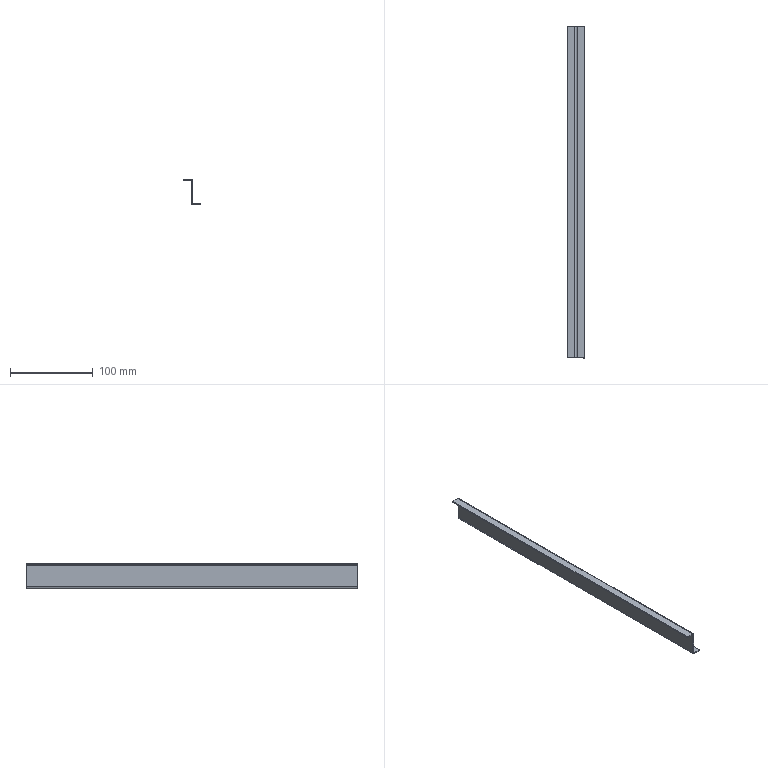Component | SolidWorks | Bracket1-6 | 1 solid | 22 faces | box 20.5 x 400 x 31 mm | volume 29099 mm3 | plane 18 | cylinder 4 | commonest cylinder face diameters 5 x2 2 x2
STEP:
#1=COLOUR_RGB('',0.7922,0.8196,0.9333);
#2=FILL_AREA_STYLE_COLOUR('',#1);
#3=FILL_AREA_STYLE('',(#2));
#4=SURFACE_STYLE_FILL_AREA(#3);
#5=SURFACE_SIDE_STYLE('',(#4));
#6=SURFACE_STYLE_USAGE(.BOTH.,#5);
#7=PRESENTATION_STYLE_ASSIGNMENT((#6));
#8=CARTESIAN_POINT('',(-9.672,3.997,61.752));
#9=VERTEX_POINT('',#8);
#10=CARTESIAN_POINT('',(-9.731,3.997,61.752));
#11=VERTEX_POINT('',#10);
#12=CARTESIAN_POINT('',(-9.672,3.997,61.752));
#13=DIRECTION('',(-1.,0.,-0.));
#14=VECTOR('',#13,39.37);
#15=LINE('',#12,#14);
#16=EDGE_CURVE('',#9,#11,#15,.T.);
#17=ORIENTED_EDGE('',*,*,#16,.F.);
#18=CARTESIAN_POINT('',(-9.633,3.997,61.713));
#19=VERTEX_POINT('',#18);
#20=CARTESIAN_POINT('',(-9.633,3.997,61.752));
#21=DIRECTION('',(0.,1.,0.));
#22=DIRECTION('',(-1.,0.,0.));
#23=AXIS2_PLACEMENT_3D('',#20,#21,#22);
#24=CIRCLE('',#23,0.03937);
#25=EDGE_CURVE('',#19,#9,#24,.T.);
#26=ORIENTED_EDGE('',*,*,#25,.F.);
#27=CARTESIAN_POINT('',(-9.633,3.997,61.654));
#28=VERTEX_POINT('',#27);
#29=CARTESIAN_POINT('',(-9.633,3.997,61.654));
#30=DIRECTION('',(-0.,-0.,1.));
#31=VECTOR('',#30,39.37);
#32=LINE('',#29,#31);
#33=EDGE_CURVE('',#28,#19,#32,.T.);
#34=ORIENTED_EDGE('',*,*,#33,.F.);
#35=CARTESIAN_POINT('',(-9.633,3.997,61.752));
#36=DIRECTION('',(0.,1.,0.));
#37=DIRECTION('',(1.,-0.,0.));
#38=AXIS2_PLACEMENT_3D('',#35,#36,#37);
#39=CIRCLE('',#38,0.09843);
#40=EDGE_CURVE('',#28,#11,#39,.T.);
#41=ORIENTED_EDGE('',*,*,#40,.T.);
#42=EDGE_LOOP('',(#17,#26,#34,#41));
#43=FACE_OUTER_BOUND('',#42,.T.);
#44=CARTESIAN_POINT('',(-9.672,3.997,61.752));
#45=DIRECTION('',(0.,1.,0.));
#46=DIRECTION('',(1.,-0.,0.));
#47=AXIS2_PLACEMENT_3D('',#44,#45,#46);
#48=PLANE('',#47);
#49=ADVANCED_FACE('',(#43),#48,.T.);
#50=CARTESIAN_POINT('',(-9.672,3.997,62.776));
#51=VERTEX_POINT('',#50);
#52=CARTESIAN_POINT('',(-9.672,3.997,62.874));
#53=DIRECTION('',(-0.,-0.,1.));
#54=VECTOR('',#53,39.37);
#55=LINE('',#52,#54);
#56=EDGE_CURVE('',#9,#51,#55,.T.);
#57=ORIENTED_EDGE('',*,*,#56,.F.);
#58=ORIENTED_EDGE('',*,*,#16,.T.);
#59=CARTESIAN_POINT('',(-9.731,3.997,62.776));
#60=VERTEX_POINT('',#59);
#61=CARTESIAN_POINT('',(-9.731,3.997,62.874));
#62=DIRECTION('',(-0.,-0.,1.));
#63=VECTOR('',#62,39.37);
#64=LINE('',#61,#63);
#65=EDGE_CURVE('',#11,#60,#64,.T.);
#66=ORIENTED_EDGE('',*,*,#65,.T.);
#67=CARTESIAN_POINT('',(-9.731,3.997,62.776));
#68=DIRECTION('',(1.,-0.,0.));
#69=VECTOR('',#68,39.37);
#70=LINE('',#67,#69);
#71=EDGE_CURVE('',#60,#51,#70,.T.);
#72=ORIENTED_EDGE('',*,*,#71,.T.);
#73=EDGE_LOOP('',(#57,#58,#66,#72));
#74=FACE_OUTER_BOUND('',#73,.T.);
#75=CARTESIAN_POINT('',(-9.633,3.997,61.654));
#76=DIRECTION('',(0.,1.,0.));
#77=DIRECTION('',(1.,-0.,0.));
#78=AXIS2_PLACEMENT_3D('',#75,#76,#77);
#79=PLANE('',#78);
#80=ADVANCED_FACE('',(#74),#79,.T.);
#81=CARTESIAN_POINT('',(-9.633,-11.751,61.713));
#82=VERTEX_POINT('',#81);
#83=CARTESIAN_POINT('',(-9.633,-11.751,61.654));
#84=VERTEX_POINT('',#83);
#85=CARTESIAN_POINT('',(-9.633,-11.751,61.713));
#86=DIRECTION('',(0.,0.,-1.));
#87=VECTOR('',#86,39.37);
#88=LINE('',#85,#87);
#89=EDGE_CURVE('',#82,#84,#88,.T.);
#90=ORIENTED_EDGE('',*,*,#89,.F.);
#91=CARTESIAN_POINT('',(-9.672,-11.751,61.752));
#92=VERTEX_POINT('',#91);
#93=CARTESIAN_POINT('',(-9.633,-11.751,61.752));
#94=DIRECTION('',(0.,1.,0.));
#95=DIRECTION('',(-1.,0.,0.));
#96=AXIS2_PLACEMENT_3D('',#93,#94,#95);
#97=CIRCLE('',#96,0.03937);
#98=EDGE_CURVE('',#82,#92,#97,.T.);
#99=ORIENTED_EDGE('',*,*,#98,.T.);
#100=CARTESIAN_POINT('',(-9.731,-11.751,61.752));
#101=VERTEX_POINT('',#100);
#102=CARTESIAN_POINT('',(-9.731,-11.751,61.752));
#103=DIRECTION('',(1.,-0.,0.));
#104=VECTOR('',#103,39.37);
#105=LINE('',#102,#104);
#106=EDGE_CURVE('',#101,#92,#105,.T.);
#107=ORIENTED_EDGE('',*,*,#106,.F.);
#108=CARTESIAN_POINT('',(-9.633,-11.751,61.752));
#109=DIRECTION('',(0.,1.,0.));
#110=DIRECTION('',(1.,0.,0.));
#111=AXIS2_PLACEMENT_3D('',#108,#109,#110);
#112=CIRCLE('',#111,0.09843);
#113=EDGE_CURVE('',#84,#101,#112,.T.);
#114=ORIENTED_EDGE('',*,*,#113,.F.);
#115=EDGE_LOOP('',(#90,#99,#107,#114));
#116=FACE_OUTER_BOUND('',#115,.T.);
#117=CARTESIAN_POINT('',(-9.633,-11.751,61.713));
#118=DIRECTION('',(-0.,-1.,-0.));
#119=DIRECTION('',(-1.,0.,-0.));
#120=AXIS2_PLACEMENT_3D('',#117,#118,#119);
#121=PLANE('',#120);
#122=ADVANCED_FACE('',(#116),#121,.T.);
#123=CARTESIAN_POINT('',(-9.298,-11.751,61.713));
#124=VERTEX_POINT('',#123);
#125=CARTESIAN_POINT('',(-9.672,-11.751,61.713));
#126=DIRECTION('',(-1.,0.,-0.));
#127=VECTOR('',#126,39.37);
#128=LINE('',#125,#127);
#129=EDGE_CURVE('',#124,#82,#128,.T.);
#130=ORIENTED_EDGE('',*,*,#129,.T.);
#131=ORIENTED_EDGE('',*,*,#89,.T.);
#132=CARTESIAN_POINT('',(-9.298,-11.751,61.654));
#133=VERTEX_POINT('',#132);
#134=CARTESIAN_POINT('',(-9.672,-11.751,61.654));
#135=DIRECTION('',(-1.,0.,-0.));
#136=VECTOR('',#135,39.37);
#137=LINE('',#134,#136);
#138=EDGE_CURVE('',#133,#84,#137,.T.);
#139=ORIENTED_EDGE('',*,*,#138,.F.);
#140=CARTESIAN_POINT('',(-9.298,-11.751,61.654));
#141=DIRECTION('',(-0.,-0.,1.));
#142=VECTOR('',#141,39.37);
#143=LINE('',#140,#142);
#144=EDGE_CURVE('',#133,#124,#143,.T.);
#145=ORIENTED_EDGE('',*,*,#144,.T.);
#146=EDGE_LOOP('',(#130,#131,#139,#145));
#147=FACE_OUTER_BOUND('',#146,.T.);
#148=CARTESIAN_POINT('',(-9.731,-11.751,61.752));
#149=DIRECTION('',(-0.,-1.,-0.));
#150=DIRECTION('',(-1.,0.,-0.));
#151=AXIS2_PLACEMENT_3D('',#148,#149,#150);
#152=PLANE('',#151);
#153=ADVANCED_FACE('',(#147),#152,.T.);
#154=CARTESIAN_POINT('',(-9.771,3.997,62.874));
#155=VERTEX_POINT('',#154);
#156=CARTESIAN_POINT('',(-9.771,3.997,62.815));
#157=VERTEX_POINT('',#156);
#158=CARTESIAN_POINT('',(-9.771,3.997,62.874));
#159=DIRECTION('',(0.,0.,-1.));
#160=VECTOR('',#159,39.37);
#161=LINE('',#158,#160);
#162=EDGE_CURVE('',#155,#157,#161,.T.);
#163=ORIENTED_EDGE('',*,*,#162,.F.);
#164=CARTESIAN_POINT('',(-9.771,3.997,62.776));
#165=DIRECTION('',(-0.,-1.,-0.));
#166=DIRECTION('',(1.,-0.,0.));
#167=AXIS2_PLACEMENT_3D('',#164,#165,#166);
#168=CIRCLE('',#167,0.09843);
#169=EDGE_CURVE('',#51,#155,#168,.T.);
#170=ORIENTED_EDGE('',*,*,#169,.F.);
#171=ORIENTED_EDGE('',*,*,#71,.F.);
#172=CARTESIAN_POINT('',(-9.771,3.997,62.776));
#173=DIRECTION('',(-0.,-1.,-0.));
#174=DIRECTION('',(1.,0.,0.));
#175=AXIS2_PLACEMENT_3D('',#172,#173,#174);
#176=CIRCLE('',#175,0.03937);
#177=EDGE_CURVE('',#60,#157,#176,.T.);
#178=ORIENTED_EDGE('',*,*,#177,.T.);
#179=EDGE_LOOP('',(#163,#170,#171,#178));
#180=FACE_OUTER_BOUND('',#179,.T.);
#181=CARTESIAN_POINT('',(-9.771,3.997,62.874));
#182=DIRECTION('',(0.,1.,0.));
#183=DIRECTION('',(1.,-0.,0.));
#184=AXIS2_PLACEMENT_3D('',#181,#182,#183);
#185=PLANE('',#184);
#186=ADVANCED_FACE('',(#180),#185,.T.);
#187=CARTESIAN_POINT('',(-10.105,3.997,62.874));
#188=VERTEX_POINT('',#187);
#189=CARTESIAN_POINT('',(-9.672,3.997,62.874));
#190=DIRECTION('',(-1.,0.,-0.));
#191=VECTOR('',#190,39.37);
#192=LINE('',#189,#191);
#193=EDGE_CURVE('',#155,#188,#192,.T.);
#194=ORIENTED_EDGE('',*,*,#193,.F.);
#195=ORIENTED_EDGE('',*,*,#162,.T.);
#196=CARTESIAN_POINT('',(-10.105,3.997,62.815));
#197=VERTEX_POINT('',#196);
#198=CARTESIAN_POINT('',(-9.672,3.997,62.815));
#199=DIRECTION('',(-1.,0.,-0.));
#200=VECTOR('',#199,39.37);
#201=LINE('',#198,#200);
#202=EDGE_CURVE('',#157,#197,#201,.T.);
#203=ORIENTED_EDGE('',*,*,#202,.T.);
#204=CARTESIAN_POINT('',(-10.105,3.997,62.874));
#205=DIRECTION('',(0.,0.,-1.));
#206=VECTOR('',#205,39.37);
#207=LINE('',#204,#206);
#208=EDGE_CURVE('',#188,#197,#207,.T.);
#209=ORIENTED_EDGE('',*,*,#208,.F.);
#210=EDGE_LOOP('',(#194,#195,#203,#209));
#211=FACE_OUTER_BOUND('',#210,.T.);
#212=CARTESIAN_POINT('',(-9.731,3.997,62.776));
#213=DIRECTION('',(0.,1.,0.));
#214=DIRECTION('',(1.,-0.,0.));
#215=AXIS2_PLACEMENT_3D('',#212,#213,#214);
#216=PLANE('',#215);
#217=ADVANCED_FACE('',(#211),#216,.T.);
#218=CARTESIAN_POINT('',(-9.672,-11.751,62.776));
#219=VERTEX_POINT('',#218);
#220=CARTESIAN_POINT('',(-9.731,-11.751,62.776));
#221=VERTEX_POINT('',#220);
#222=CARTESIAN_POINT('',(-9.672,-11.751,62.776));
#223=DIRECTION('',(-1.,0.,-0.));
#224=VECTOR('',#223,39.37);
#225=LINE('',#222,#224);
#226=EDGE_CURVE('',#219,#221,#225,.T.);
#227=ORIENTED_EDGE('',*,*,#226,.F.);
#228=CARTESIAN_POINT('',(-9.771,-11.751,62.874));
#229=VERTEX_POINT('',#228);
#230=CARTESIAN_POINT('',(-9.771,-11.751,62.776));
#231=DIRECTION('',(-0.,-1.,-0.));
#232=DIRECTION('',(1.,0.,0.));
#233=AXIS2_PLACEMENT_3D('',#230,#231,#232);
#234=CIRCLE('',#233,0.09843);
#235=EDGE_CURVE('',#219,#229,#234,.T.);
#236=ORIENTED_EDGE('',*,*,#235,.T.);
#237=CARTESIAN_POINT('',(-9.771,-11.751,62.815));
#238=VERTEX_POINT('',#237);
#239=CARTESIAN_POINT('',(-9.771,-11.751,62.815));
#240=DIRECTION('',(-0.,-0.,1.));
#241=VECTOR('',#240,39.37);
#242=LINE('',#239,#241);
#243=EDGE_CURVE('',#238,#229,#242,.T.);
#244=ORIENTED_EDGE('',*,*,#243,.F.);
#245=CARTESIAN_POINT('',(-9.771,-11.751,62.776));
#246=DIRECTION('',(-0.,-1.,-0.));
#247=DIRECTION('',(1.,0.,0.));
#248=AXIS2_PLACEMENT_3D('',#245,#246,#247);
#249=CIRCLE('',#248,0.03937);
#250=EDGE_CURVE('',#221,#238,#249,.T.);
#251=ORIENTED_EDGE('',*,*,#250,.F.);
#252=EDGE_LOOP('',(#227,#236,#244,#251));
#253=FACE_OUTER_BOUND('',#252,.T.);
#254=CARTESIAN_POINT('',(-9.672,-11.751,62.776));
#255=DIRECTION('',(-0.,-1.,-0.));
#256=DIRECTION('',(-1.,0.,-0.));
#257=AXIS2_PLACEMENT_3D('',#254,#255,#256);
#258=PLANE('',#257);
#259=ADVANCED_FACE('',(#253),#258,.T.);
#260=CARTESIAN_POINT('',(-9.672,-11.751,62.874));
#261=DIRECTION('',(-0.,-0.,1.));
#262=VECTOR('',#261,39.37);
#263=LINE('',#260,#262);
#264=EDGE_CURVE('',#92,#219,#263,.T.);
#265=ORIENTED_EDGE('',*,*,#264,.T.);
#266=ORIENTED_EDGE('',*,*,#226,.T.);
#267=CARTESIAN_POINT('',(-9.731,-11.751,62.874));
#268=DIRECTION('',(-0.,-0.,1.));
#269=VECTOR('',#268,39.37);
#270=LINE('',#267,#269);
#271=EDGE_CURVE('',#101,#221,#270,.T.);
#272=ORIENTED_EDGE('',*,*,#271,.F.);
#273=ORIENTED_EDGE('',*,*,#106,.T.);
#274=EDGE_LOOP('',(#265,#266,#272,#273));
#275=FACE_OUTER_BOUND('',#274,.T.);
#276=CARTESIAN_POINT('',(-9.771,-11.751,62.815));
#277=DIRECTION('',(-0.,-1.,-0.));
#278=DIRECTION('',(-1.,0.,-0.));
#279=AXIS2_PLACEMENT_3D('',#276,#277,#278);
#280=PLANE('',#279);
#281=ADVANCED_FACE('',(#275),#280,.T.);
#282=CARTESIAN_POINT('',(-10.105,-11.751,62.815));
#283=VERTEX_POINT('',#282);
#284=CARTESIAN_POINT('',(-9.672,-11.751,62.815));
#285=DIRECTION('',(-1.,0.,-0.));
#286=VECTOR('',#285,39.37);
#287=LINE('',#284,#286);
#288=EDGE_CURVE('',#238,#283,#287,.T.);
#289=ORIENTED_EDGE('',*,*,#288,.T.);
#290=CARTESIAN_POINT('',(-10.105,3.997,62.815));
#291=DIRECTION('',(-0.,-1.,-0.));
#292=VECTOR('',#291,39.37);
#293=LINE('',#290,#292);
#294=EDGE_CURVE('',#197,#283,#293,.T.);
#295=ORIENTED_EDGE('',*,*,#294,.F.);
#296=ORIENTED_EDGE('',*,*,#202,.F.);
#297=CARTESIAN_POINT('',(-9.771,3.997,62.815));
#298=DIRECTION('',(-0.,-1.,-0.));
#299=VECTOR('',#298,39.37);
#300=LINE('',#297,#299);
#301=EDGE_CURVE('',#157,#238,#300,.T.);
#302=ORIENTED_EDGE('',*,*,#301,.T.);
#303=EDGE_LOOP('',(#289,#295,#296,#302));
#304=FACE_OUTER_BOUND('',#303,.T.);
#305=CARTESIAN_POINT('',(-9.672,3.997,62.815));
#306=DIRECTION('',(-0.,-0.,1.));
#307=DIRECTION('',(1.,-0.,0.));
#308=AXIS2_PLACEMENT_3D('',#305,#306,#307);
#309=PLANE('',#308);
#310=ADVANCED_FACE('',(#304),#309,.F.);
#311=CARTESIAN_POINT('',(-10.105,-11.751,62.874));
#312=VERTEX_POINT('',#311);
#313=CARTESIAN_POINT('',(-10.105,-11.751,62.874));
#314=DIRECTION('',(0.,0.,-1.));
#315=VECTOR('',#314,39.37);
#316=LINE('',#313,#315);
#317=EDGE_CURVE('',#312,#283,#316,.T.);
#318=ORIENTED_EDGE('',*,*,#317,.F.);
#319=CARTESIAN_POINT('',(-10.105,3.997,62.874));
#320=DIRECTION('',(-0.,-1.,-0.));
#321=VECTOR('',#320,39.37);
#322=LINE('',#319,#321);
#323=EDGE_CURVE('',#188,#312,#322,.T.);
#324=ORIENTED_EDGE('',*,*,#323,.F.);
#325=ORIENTED_EDGE('',*,*,#208,.T.);
#326=ORIENTED_EDGE('',*,*,#294,.T.);
#327=EDGE_LOOP('',(#318,#324,#325,#326));
#328=FACE_OUTER_BOUND('',#327,.T.);
#329=CARTESIAN_POINT('',(-10.105,3.997,62.874));
#330=DIRECTION('',(-1.,0.,-0.));
#331=DIRECTION('',(0.,1.,0.));
#332=AXIS2_PLACEMENT_3D('',#329,#330,#331);
#333=PLANE('',#332);
#334=ADVANCED_FACE('',(#328),#333,.T.);
#335=CARTESIAN_POINT('',(-9.672,-11.751,62.874));
#336=DIRECTION('',(-1.,0.,-0.));
#337=VECTOR('',#336,39.37);
#338=LINE('',#335,#337);
#339=EDGE_CURVE('',#229,#312,#338,.T.);
#340=ORIENTED_EDGE('',*,*,#339,.F.);
#341=CARTESIAN_POINT('',(-9.771,3.997,62.874));
#342=DIRECTION('',(-0.,-1.,-0.));
#343=VECTOR('',#342,39.37);
#344=LINE('',#341,#343);
#345=EDGE_CURVE('',#155,#229,#344,.T.);
#346=ORIENTED_EDGE('',*,*,#345,.F.);
#347=ORIENTED_EDGE('',*,*,#193,.T.);
#348=ORIENTED_EDGE('',*,*,#323,.T.);
#349=EDGE_LOOP('',(#340,#346,#347,#348));
#350=FACE_OUTER_BOUND('',#349,.T.);
#351=CARTESIAN_POINT('',(-9.672,3.997,62.874));
#352=DIRECTION('',(-0.,-0.,1.));
#353=DIRECTION('',(1.,-0.,0.));
#354=AXIS2_PLACEMENT_3D('',#351,#352,#353);
#355=PLANE('',#354);
#356=ADVANCED_FACE('',(#350),#355,.T.);
#357=ORIENTED_EDGE('',*,*,#235,.F.);
#358=CARTESIAN_POINT('',(-9.672,3.997,62.776));
#359=DIRECTION('',(-0.,-1.,-0.));
#360=VECTOR('',#359,39.37);
#361=LINE('',#358,#360);
#362=EDGE_CURVE('',#51,#219,#361,.T.);
#363=ORIENTED_EDGE('',*,*,#362,.F.);
#364=ORIENTED_EDGE('',*,*,#169,.T.);
#365=ORIENTED_EDGE('',*,*,#345,.T.);
#366=EDGE_LOOP('',(#357,#363,#364,#365));
#367=FACE_OUTER_BOUND('',#366,.T.);
#368=CARTESIAN_POINT('',(-9.771,3.997,62.776));
#369=DIRECTION('',(-0.,-1.,-0.));
#370=DIRECTION('',(-1.,0.,0.));
#371=AXIS2_PLACEMENT_3D('',#368,#369,#370);
#372=CYLINDRICAL_SURFACE('',#371,0.09843);
#373=ADVANCED_FACE('',(#367),#372,.T.);
#374=ORIENTED_EDGE('',*,*,#264,.F.);
#375=CARTESIAN_POINT('',(-9.672,3.997,61.752));
#376=DIRECTION('',(-0.,-1.,-0.));
#377=VECTOR('',#376,39.37);
#378=LINE('',#375,#377);
#379=EDGE_CURVE('',#9,#92,#378,.T.);
#380=ORIENTED_EDGE('',*,*,#379,.F.);
#381=ORIENTED_EDGE('',*,*,#56,.T.);
#382=ORIENTED_EDGE('',*,*,#362,.T.);
#383=EDGE_LOOP('',(#374,#380,#381,#382));
#384=FACE_OUTER_BOUND('',#383,.T.);
#385=CARTESIAN_POINT('',(-9.672,3.997,62.874));
#386=DIRECTION('',(1.,-0.,0.));
#387=DIRECTION('',(-0.,-1.,-0.));
#388=AXIS2_PLACEMENT_3D('',#385,#386,#387);
#389=PLANE('',#388);
#390=ADVANCED_FACE('',(#384),#389,.T.);
#391=ORIENTED_EDGE('',*,*,#98,.F.);
#392=CARTESIAN_POINT('',(-9.633,3.997,61.713));
#393=DIRECTION('',(-0.,-1.,-0.));
#394=VECTOR('',#393,39.37);
#395=LINE('',#392,#394);
#396=EDGE_CURVE('',#19,#82,#395,.T.);
#397=ORIENTED_EDGE('',*,*,#396,.F.);
#398=ORIENTED_EDGE('',*,*,#25,.T.);
#399=ORIENTED_EDGE('',*,*,#379,.T.);
#400=EDGE_LOOP('',(#391,#397,#398,#399));
#401=FACE_OUTER_BOUND('',#400,.T.);
#402=CARTESIAN_POINT('',(-9.633,3.997,61.752));
#403=DIRECTION('',(-0.,-1.,-0.));
#404=DIRECTION('',(-1.,0.,0.));
#405=AXIS2_PLACEMENT_3D('',#402,#403,#404);
#406=CYLINDRICAL_SURFACE('',#405,0.03937);
#407=ADVANCED_FACE('',(#401),#406,.F.);
#408=ORIENTED_EDGE('',*,*,#129,.F.);
#409=CARTESIAN_POINT('',(-9.298,3.997,61.713));
#410=VERTEX_POINT('',#409);
#411=CARTESIAN_POINT('',(-9.298,3.997,61.713));
#412=DIRECTION('',(-0.,-1.,-0.));
#413=VECTOR('',#412,39.37);
#414=LINE('',#411,#413);
#415=EDGE_CURVE('',#410,#124,#414,.T.);
#416=ORIENTED_EDGE('',*,*,#415,.F.);
#417=CARTESIAN_POINT('',(-9.672,3.997,61.713));
#418=DIRECTION('',(-1.,0.,-0.));
#419=VECTOR('',#418,39.37);
#420=LINE('',#417,#419);
#421=EDGE_CURVE('',#410,#19,#420,.T.);
#422=ORIENTED_EDGE('',*,*,#421,.T.);
#423=ORIENTED_EDGE('',*,*,#396,.T.);
#424=EDGE_LOOP('',(#408,#416,#422,#423));
#425=FACE_OUTER_BOUND('',#424,.T.);
#426=CARTESIAN_POINT('',(-9.672,3.997,61.713));
#427=DIRECTION('',(-0.,-0.,1.));
#428=DIRECTION('',(-0.,-1.,-0.));
#429=AXIS2_PLACEMENT_3D('',#426,#427,#428);
#430=PLANE('',#429);
#431=ADVANCED_FACE('',(#425),#430,.T.);
#432=ORIENTED_EDGE('',*,*,#144,.F.);
#433=CARTESIAN_POINT('',(-9.298,3.997,61.654));
#434=VERTEX_POINT('',#433);
#435=CARTESIAN_POINT('',(-9.298,3.997,61.654));
#436=DIRECTION('',(-0.,-1.,-0.));
#437=VECTOR('',#436,39.37);
#438=LINE('',#435,#437);
#439=EDGE_CURVE('',#434,#133,#438,.T.);
#440=ORIENTED_EDGE('',*,*,#439,.F.);
#441=CARTESIAN_POINT('',(-9.298,3.997,61.654));
#442=DIRECTION('',(-0.,-0.,1.));
#443=VECTOR('',#442,39.37);
#444=LINE('',#441,#443);
#445=EDGE_CURVE('',#434,#410,#444,.T.);
#446=ORIENTED_EDGE('',*,*,#445,.T.);
#447=ORIENTED_EDGE('',*,*,#415,.T.);
#448=EDGE_LOOP('',(#432,#440,#446,#447));
#449=FACE_OUTER_BOUND('',#448,.T.);
#450=CARTESIAN_POINT('',(-9.298,3.997,61.654));
#451=DIRECTION('',(1.,-0.,0.));
#452=DIRECTION('',(-0.,-1.,-0.));
#453=AXIS2_PLACEMENT_3D('',#450,#451,#452);
#454=PLANE('',#453);
#455=ADVANCED_FACE('',(#449),#454,.T.);
#456=ORIENTED_EDGE('',*,*,#138,.T.);
#457=CARTESIAN_POINT('',(-9.633,3.997,61.654));
#458=DIRECTION('',(-0.,-1.,-0.));
#459=VECTOR('',#458,39.37);
#460=LINE('',#457,#459);
#461=EDGE_CURVE('',#28,#84,#460,.T.);
#462=ORIENTED_EDGE('',*,*,#461,.F.);
#463=CARTESIAN_POINT('',(-9.672,3.997,61.654));
#464=DIRECTION('',(-1.,0.,-0.));
#465=VECTOR('',#464,39.37);
#466=LINE('',#463,#465);
#467=EDGE_CURVE('',#434,#28,#466,.T.);
#468=ORIENTED_EDGE('',*,*,#467,.F.);
#469=ORIENTED_EDGE('',*,*,#439,.T.);
#470=EDGE_LOOP('',(#456,#462,#468,#469));
#471=FACE_OUTER_BOUND('',#470,.T.);
#472=CARTESIAN_POINT('',(-9.672,3.997,61.654));
#473=DIRECTION('',(-0.,-0.,1.));
#474=DIRECTION('',(-0.,-1.,-0.));
#475=AXIS2_PLACEMENT_3D('',#472,#473,#474);
#476=PLANE('',#475);
#477=ADVANCED_FACE('',(#471),#476,.F.);
#478=ORIENTED_EDGE('',*,*,#113,.T.);
#479=CARTESIAN_POINT('',(-9.731,3.997,61.752));
#480=DIRECTION('',(-0.,-1.,-0.));
#481=VECTOR('',#480,39.37);
#482=LINE('',#479,#481);
#483=EDGE_CURVE('',#11,#101,#482,.T.);
#484=ORIENTED_EDGE('',*,*,#483,.F.);
#485=ORIENTED_EDGE('',*,*,#40,.F.);
#486=ORIENTED_EDGE('',*,*,#461,.T.);
#487=EDGE_LOOP('',(#478,#484,#485,#486));
#488=FACE_OUTER_BOUND('',#487,.T.);
#489=CARTESIAN_POINT('',(-9.633,3.997,61.752));
#490=DIRECTION('',(-0.,-1.,-0.));
#491=DIRECTION('',(-1.,0.,0.));
#492=AXIS2_PLACEMENT_3D('',#489,#490,#491);
#493=CYLINDRICAL_SURFACE('',#492,0.09843);
#494=ADVANCED_FACE('',(#488),#493,.T.);
#495=ORIENTED_EDGE('',*,*,#271,.T.);
#496=CARTESIAN_POINT('',(-9.731,3.997,62.776));
#497=DIRECTION('',(-0.,-1.,-0.));
#498=VECTOR('',#497,39.37);
#499=LINE('',#496,#498);
#500=EDGE_CURVE('',#60,#221,#499,.T.);
#501=ORIENTED_EDGE('',*,*,#500,.F.);
#502=ORIENTED_EDGE('',*,*,#65,.F.);
#503=ORIENTED_EDGE('',*,*,#483,.T.);
#504=EDGE_LOOP('',(#495,#501,#502,#503));
#505=FACE_OUTER_BOUND('',#504,.T.);
#506=CARTESIAN_POINT('',(-9.731,3.997,62.874));
#507=DIRECTION('',(1.,-0.,0.));
#508=DIRECTION('',(-0.,-1.,-0.));
#509=AXIS2_PLACEMENT_3D('',#506,#507,#508);
#510=PLANE('',#509);
#511=ADVANCED_FACE('',(#505),#510,.F.);
#512=ORIENTED_EDGE('',*,*,#250,.T.);
#513=ORIENTED_EDGE('',*,*,#301,.F.);
#514=ORIENTED_EDGE('',*,*,#177,.F.);
#515=ORIENTED_EDGE('',*,*,#500,.T.);
#516=EDGE_LOOP('',(#512,#513,#514,#515));
#517=FACE_OUTER_BOUND('',#516,.T.);
#518=CARTESIAN_POINT('',(-9.771,3.997,62.776));
#519=DIRECTION('',(-0.,-1.,-0.));
#520=DIRECTION('',(-1.,0.,0.));
#521=AXIS2_PLACEMENT_3D('',#518,#519,#520);
#522=CYLINDRICAL_SURFACE('',#521,0.03937);
#523=ADVANCED_FACE('',(#517),#522,.F.);
#524=ORIENTED_EDGE('',*,*,#467,.T.);
#525=ORIENTED_EDGE('',*,*,#33,.T.);
#526=ORIENTED_EDGE('',*,*,#421,.F.);
#527=ORIENTED_EDGE('',*,*,#445,.F.);
#528=EDGE_LOOP('',(#524,#525,#526,#527));
#529=FACE_OUTER_BOUND('',#528,.T.);
#530=CARTESIAN_POINT('',(-9.771,3.997,62.776));
#531=DIRECTION('',(0.,1.,0.));
#532=DIRECTION('',(1.,-0.,0.));
#533=AXIS2_PLACEMENT_3D('',#530,#531,#532);
#534=PLANE('',#533);
#535=ADVANCED_FACE('',(#529),#534,.T.);
#536=ORIENTED_EDGE('',*,*,#288,.F.);
#537=ORIENTED_EDGE('',*,*,#243,.T.);
#538=ORIENTED_EDGE('',*,*,#339,.T.);
#539=ORIENTED_EDGE('',*,*,#317,.T.);
#540=EDGE_LOOP('',(#536,#537,#538,#539));
#541=FACE_OUTER_BOUND('',#540,.T.);
#542=CARTESIAN_POINT('',(-9.771,-11.751,62.776));
#543=DIRECTION('',(0.,1.,0.));
#544=DIRECTION('',(1.,-0.,0.));
#545=AXIS2_PLACEMENT_3D('',#542,#543,#544);
#546=PLANE('',#545);
#547=ADVANCED_FACE('',(#541),#546,.F.);
#548=CLOSED_SHELL('',(#49,#80,#122,#153,#186,#217,#259,#281,#310,#334,#356,#373,#390,#407,#431,#455,#477,#494,#511,#523,#535,#547));
#549=MANIFOLD_SOLID_BREP('',#548);
#550=STYLED_ITEM('',(#7),#549);
#551=(LENGTH_UNIT()NAMED_UNIT(*)SI_UNIT($,.METRE.));
#552=LENGTH_MEASURE_WITH_UNIT(LENGTH_MEASURE(0.0254),#551);
#553=DIMENSIONAL_EXPONENTS(1.,0.,0.,0.,0.,0.,0.);
#554=(CONVERSION_BASED_UNIT('',#552)LENGTH_UNIT()NAMED_UNIT(#553));
#555=UNCERTAINTY_MEASURE_WITH_UNIT(LENGTH_MEASURE(0.00001),#554,'','');
#556=(NAMED_UNIT(*)PLANE_ANGLE_UNIT()SI_UNIT($,.RADIAN.));
#557=(NAMED_UNIT(*)SI_UNIT($,.STERADIAN.)SOLID_ANGLE_UNIT());
#558=(GEOMETRIC_REPRESENTATION_CONTEXT(3)GLOBAL_UNCERTAINTY_ASSIGNED_CONTEXT((#555))GLOBAL_UNIT_ASSIGNED_CONTEXT((#554,#556,#557))REPRESENTATION_CONTEXT('',''));
#559=MECHANICAL_DESIGN_GEOMETRIC_PRESENTATION_REPRESENTATION('',(#550),#558);
#560=CARTESIAN_POINT('',(0.,0.,0.));
#561=DIRECTION('',(0.,0.,1.));
#562=DIRECTION('',(1.,0.,0.));
#563=AXIS2_PLACEMENT_3D('',#560,#561,#562);
#564=(LENGTH_UNIT()NAMED_UNIT(*)SI_UNIT($,.METRE.));
#565=LENGTH_MEASURE_WITH_UNIT(LENGTH_MEASURE(0.0254),#564);
#566=DIMENSIONAL_EXPONENTS(1.,0.,0.,0.,0.,0.,0.);
#567=(CONVERSION_BASED_UNIT('',#565)LENGTH_UNIT()NAMED_UNIT(#566));
#568=UNCERTAINTY_MEASURE_WITH_UNIT(LENGTH_MEASURE(0.00001),#567,'','');
#569=(NAMED_UNIT(*)PLANE_ANGLE_UNIT()SI_UNIT($,.RADIAN.));
#570=(NAMED_UNIT(*)SI_UNIT($,.STERADIAN.)SOLID_ANGLE_UNIT());
#571=(GEOMETRIC_REPRESENTATION_CONTEXT(3)GLOBAL_UNCERTAINTY_ASSIGNED_CONTEXT((#568))GLOBAL_UNIT_ASSIGNED_CONTEXT((#567,#569,#570))REPRESENTATION_CONTEXT('',''));
#572=ADVANCED_BREP_SHAPE_REPRESENTATION('',(#549,#563),#571);
#573=PRESENTATION_LAYER_ASSIGNMENT('','',(#550));